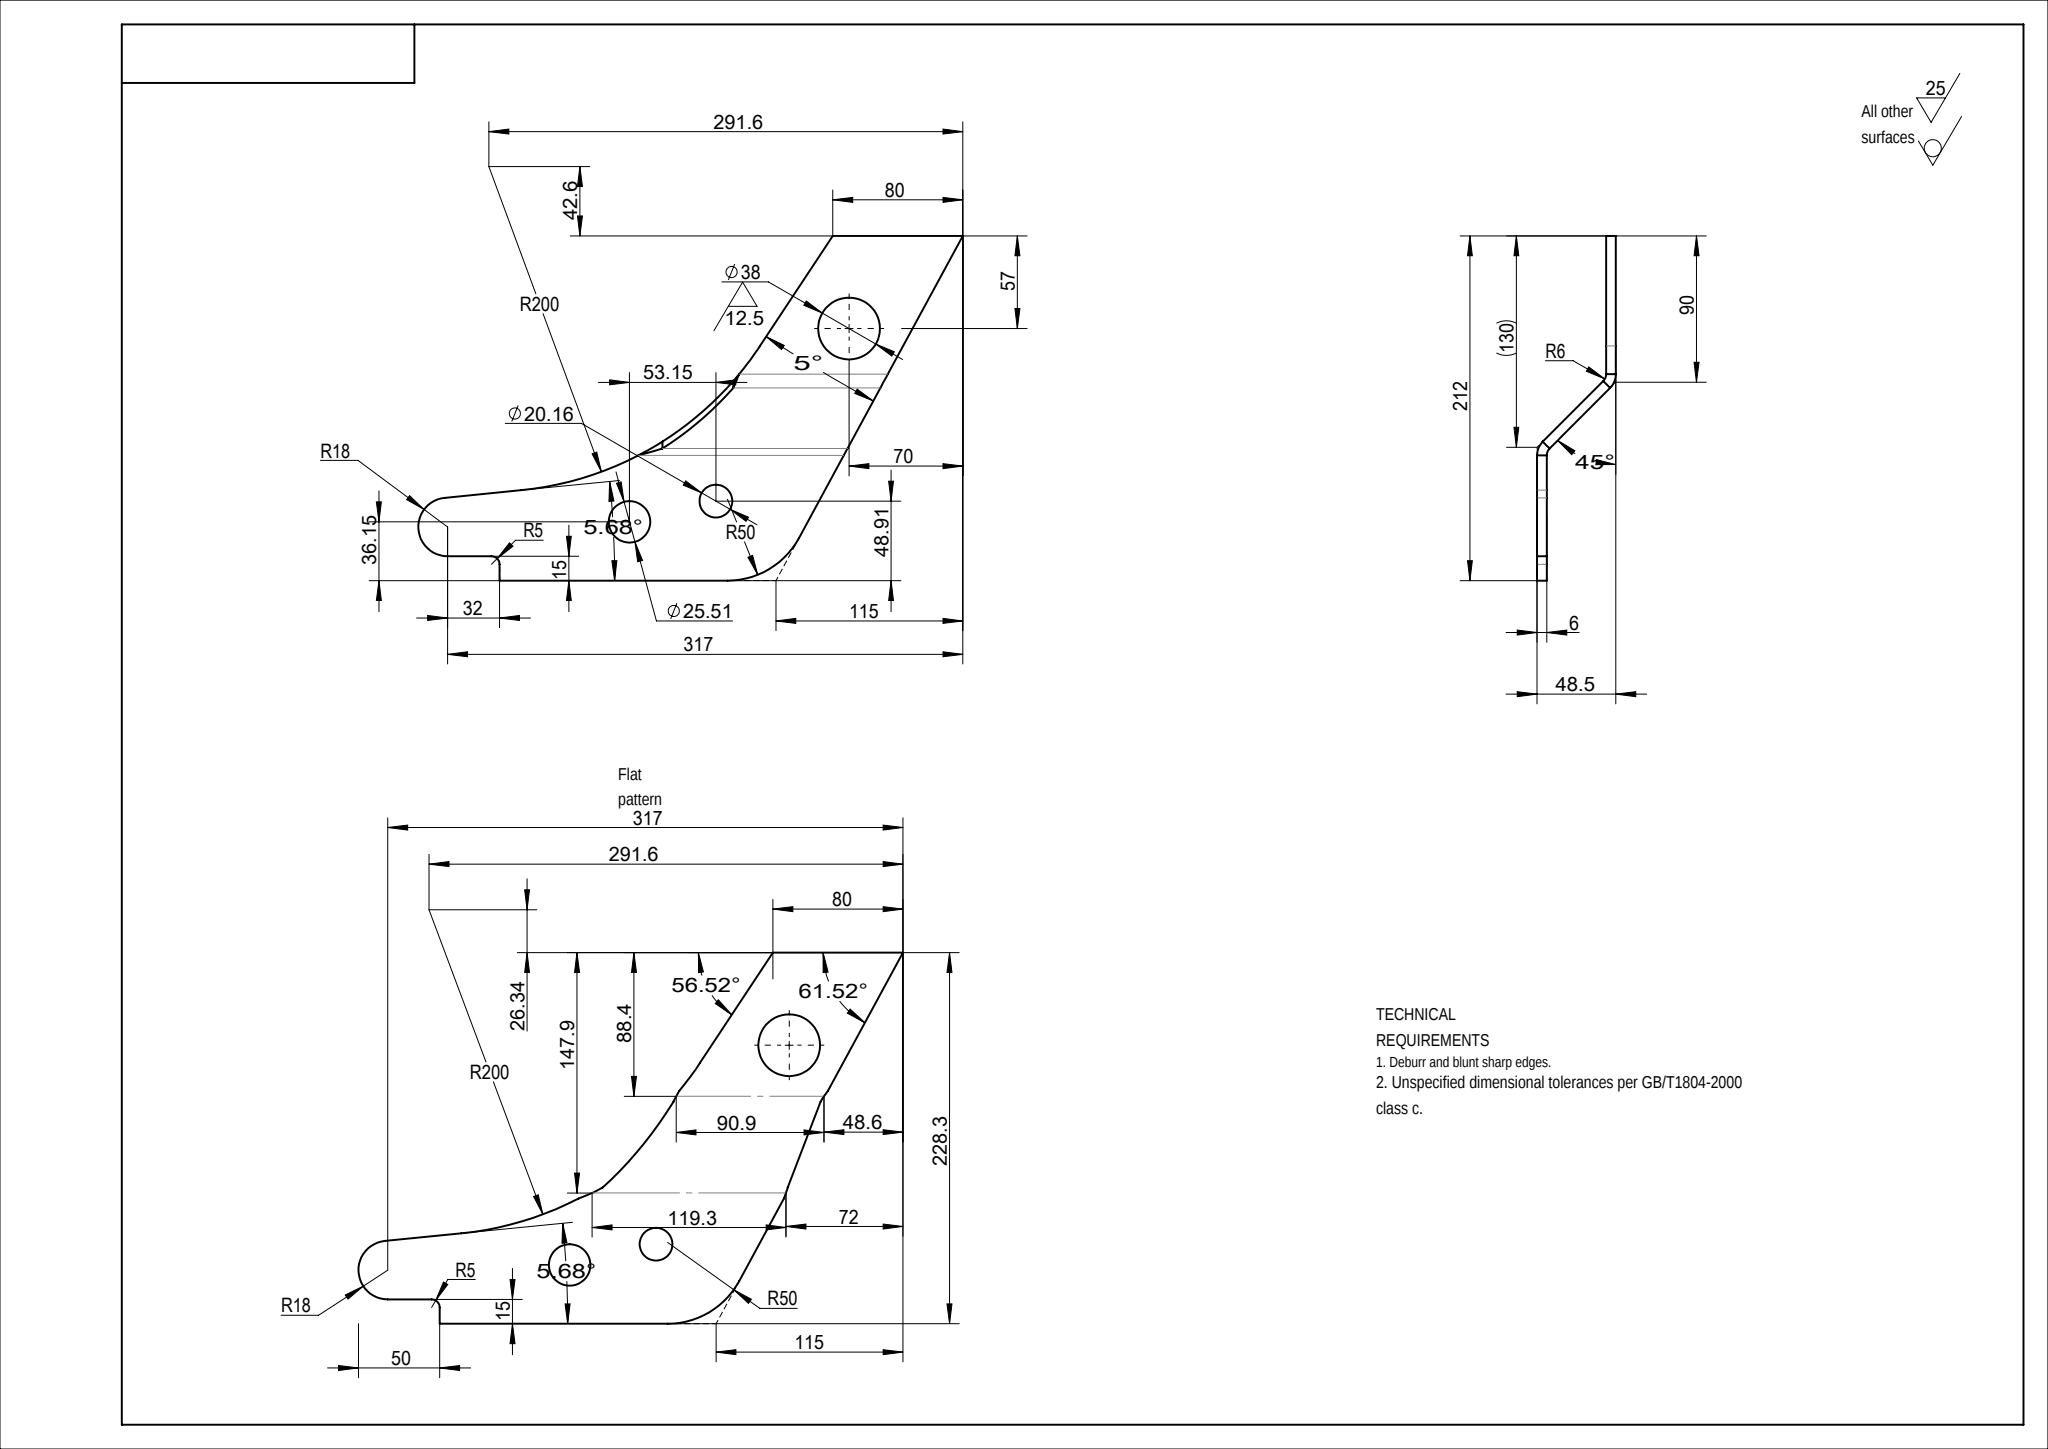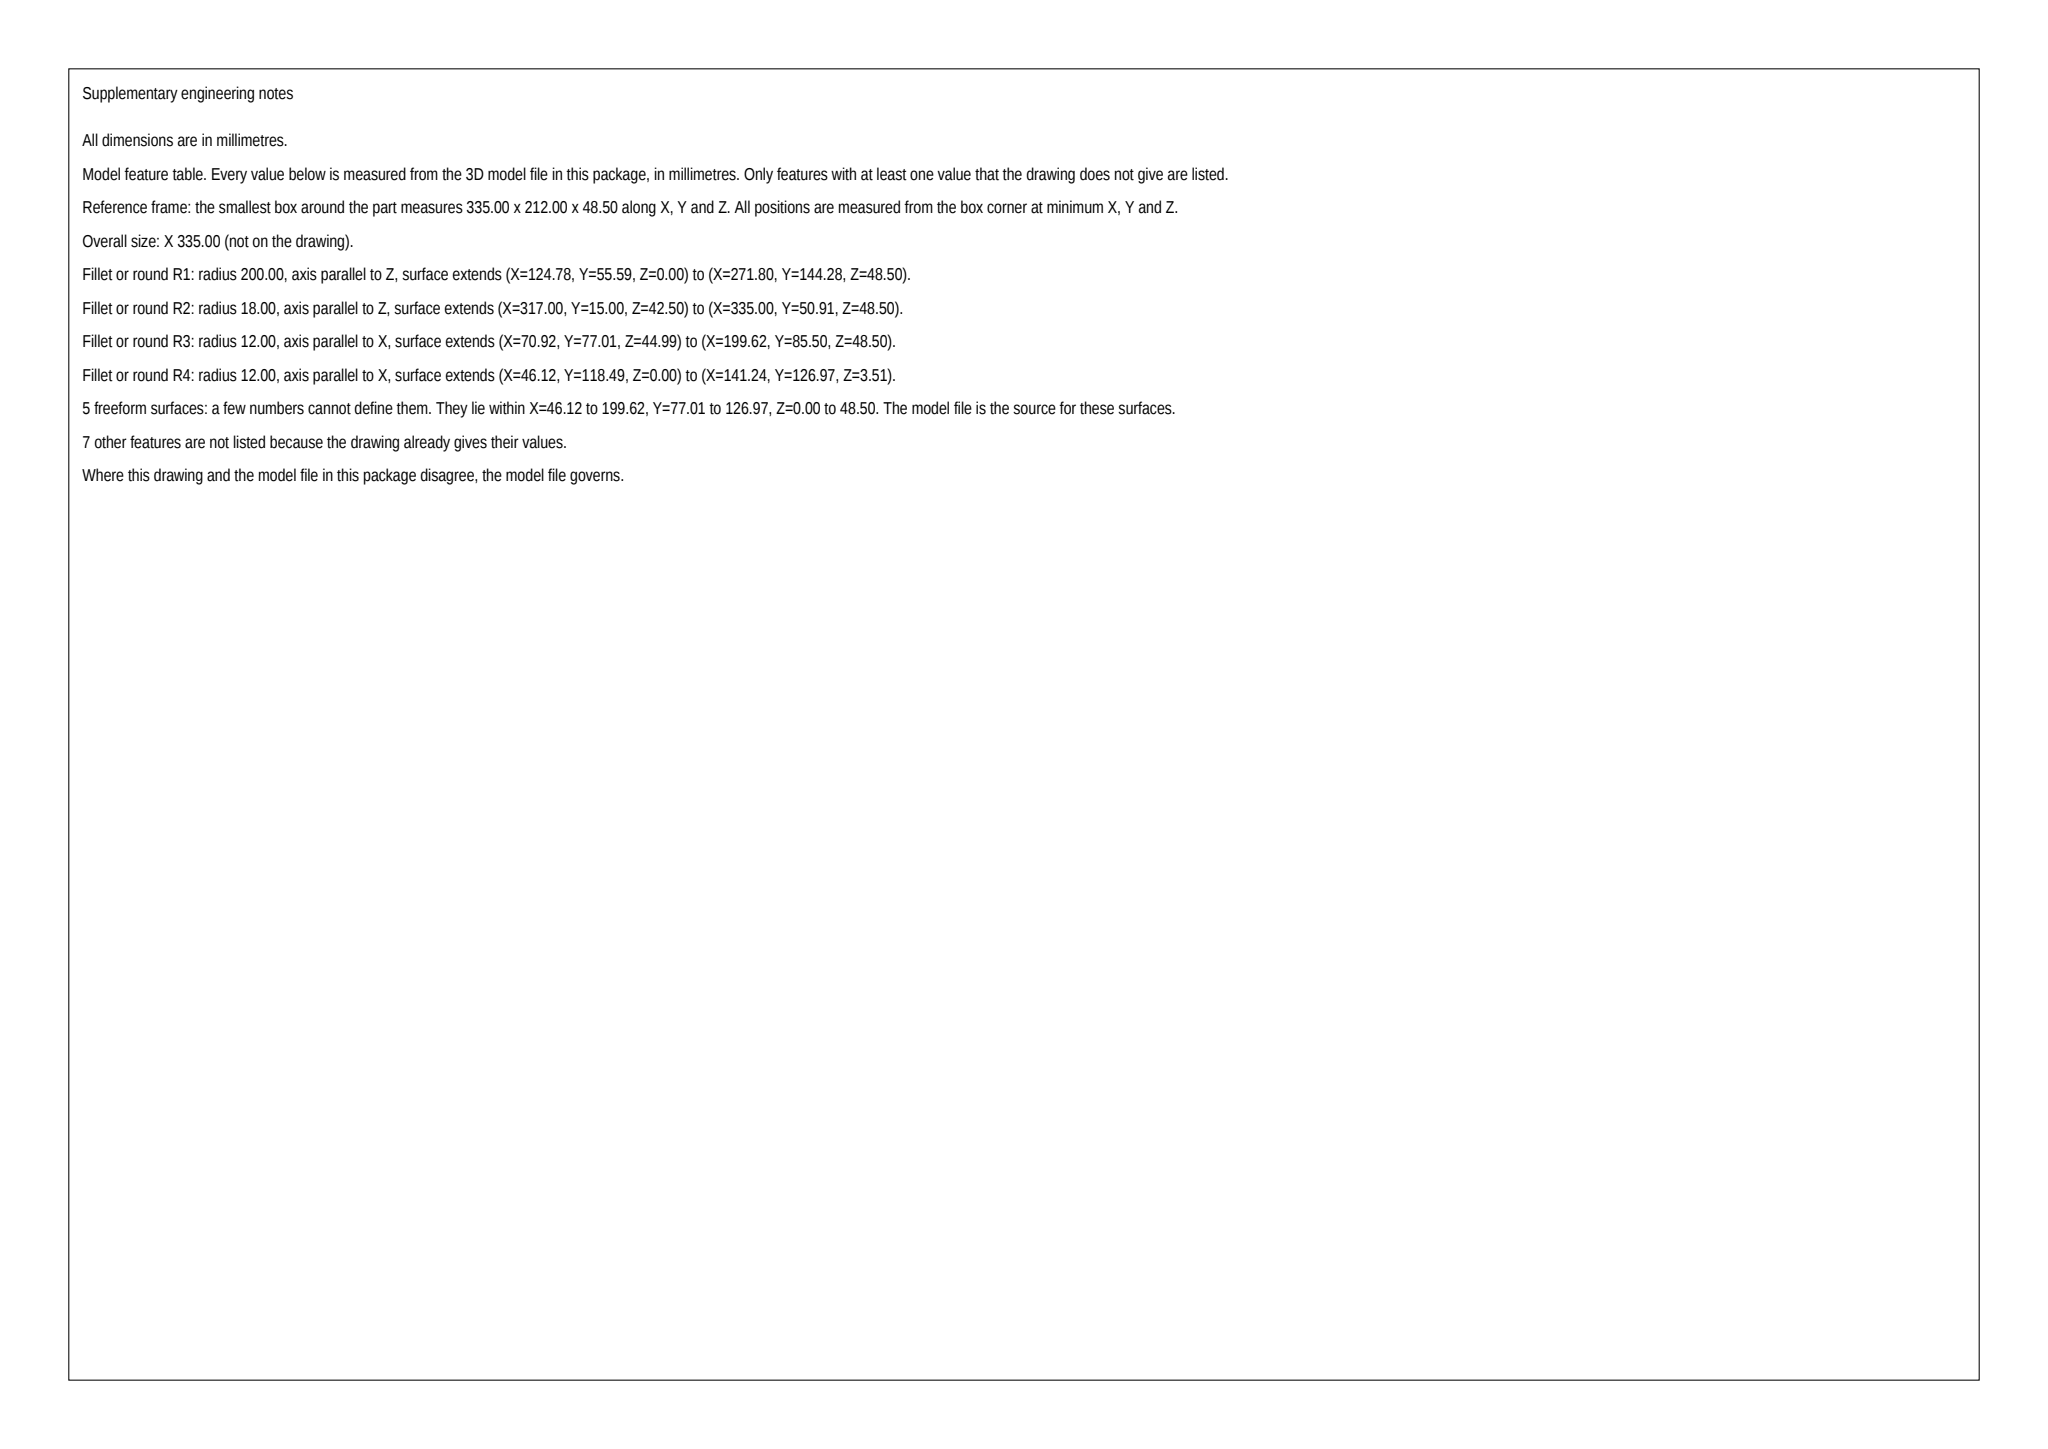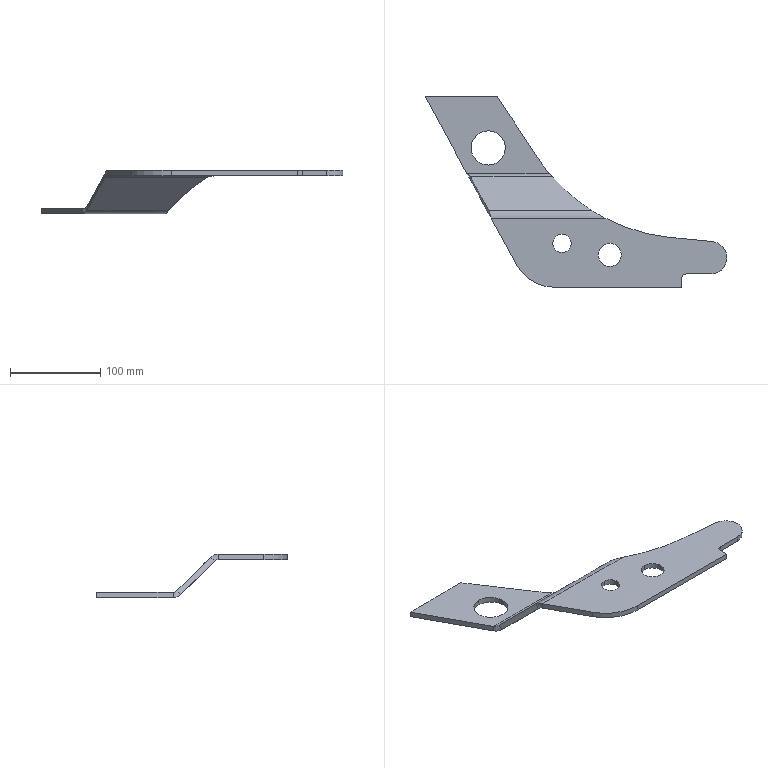Part | SolidWorks | mm | 1 solid | 35 faces | box 335 x 212 x 48.5 mm | volume 162382 mm3 | cylinder 15 | plane 15 | spline 5 | commonest cylinder face diameters 25.511 x2 24 x2 12 x2 400 x2 38 x2 20.161 x2 36 x1 10 x1